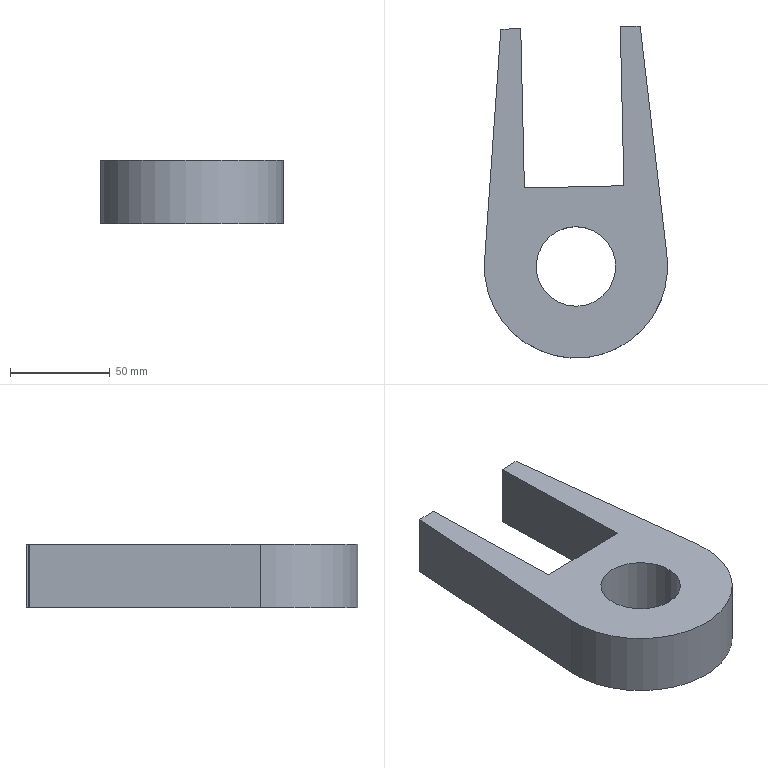Component | NX | 11 | 1 solid | 11 faces | box 92 x 166.77 x 32 mm | volume 249939 mm3 | plane 9 | cylinder 2 | commonest cylinder face diameters 92 x1 40 x1
STEP:
#1=CARTESIAN_POINT('',(0.,0.,0.));
#2=DIRECTION('',(0.,0.,1.));
#3=DIRECTION('',(1.,0.,0.));
#4=AXIS2_PLACEMENT_3D('',#1,#2,#3);
#5=CARTESIAN_POINT('',(-323.626,-1050.37,184.288));
#6=VERTEX_POINT('',#5);
#7=CARTESIAN_POINT('',(-313.628,-1050.142,184.288));
#8=VERTEX_POINT('',#7);
#9=CARTESIAN_POINT('',(-323.626,-1050.37,184.288));
#10=DIRECTION('',(0.9997,0.02285,0.));
#11=VECTOR('',#10,1.);
#12=LINE('',#9,#11);
#13=CARTESIAN_POINT('',(-323.626,-1050.37,152.288));
#14=DIRECTION('',(0.02285,-0.9997,0.));
#15=DIRECTION('',(-0.9997,-0.02285,0.));
#16=AXIS2_PLACEMENT_3D('',#13,#14,#15);
#17=PLANE('',#16);
#18=CARTESIAN_POINT('',(0.,-32.));
#19=DIRECTION('',(-1.,0.));
#20=VECTOR('',#19,1.);
#21=LINE('',#18,#20);
#22=(GEOMETRIC_REPRESENTATION_CONTEXT(2)PARAMETRIC_REPRESENTATION_CONTEXT()REPRESENTATION_CONTEXT('',''));
#23=DEFINITIONAL_REPRESENTATION('',(#21),#22);
#24=PCURVE('',#17,#23);
#25=CARTESIAN_POINT('',(-345.877,-1170.91,184.288));
#26=DIRECTION('',(0.,0.,-1.));
#27=DIRECTION('',(0.9997,0.02285,0.));
#28=AXIS2_PLACEMENT_3D('',#25,#26,#27);
#29=PLANE('',#28);
#30=CARTESIAN_POINT('',(25.,-120.));
#31=DIRECTION('',(1.,0.));
#32=VECTOR('',#31,1.);
#33=LINE('',#30,#32);
#34=(GEOMETRIC_REPRESENTATION_CONTEXT(2)PARAMETRIC_REPRESENTATION_CONTEXT()REPRESENTATION_CONTEXT('',''));
#35=DEFINITIONAL_REPRESENTATION('',(#33),#34);
#36=PCURVE('',#29,#35);
#37=SURFACE_CURVE('',#12,(#24,#36),.PCURVE_S1.);
#38=EDGE_CURVE('',#6,#8,#37,.T.);
#39=ORIENTED_EDGE('',*,*,#38,.T.);
#40=CARTESIAN_POINT('',(-313.628,-1050.142,152.288));
#41=VERTEX_POINT('',#40);
#42=CARTESIAN_POINT('',(-313.628,-1050.142,152.288));
#43=DIRECTION('',(0.,0.,1.));
#44=VECTOR('',#43,1.);
#45=LINE('',#42,#44);
#46=CARTESIAN_POINT('',(-10.,0.));
#47=DIRECTION('',(0.,-1.));
#48=VECTOR('',#47,1.);
#49=LINE('',#46,#48);
#50=(GEOMETRIC_REPRESENTATION_CONTEXT(2)PARAMETRIC_REPRESENTATION_CONTEXT()REPRESENTATION_CONTEXT('',''));
#51=DEFINITIONAL_REPRESENTATION('',(#49),#50);
#52=PCURVE('',#17,#51);
#53=CARTESIAN_POINT('',(-313.628,-1050.142,152.288));
#54=DIRECTION('',(-0.9933,-0.1157,0.));
#55=DIRECTION('',(-0.1157,0.9933,0.));
#56=AXIS2_PLACEMENT_3D('',#53,#54,#55);
#57=PLANE('',#56);
#58=CARTESIAN_POINT('',(0.,0.));
#59=DIRECTION('',(0.,-1.));
#60=VECTOR('',#59,1.);
#61=LINE('',#58,#60);
#62=(GEOMETRIC_REPRESENTATION_CONTEXT(2)PARAMETRIC_REPRESENTATION_CONTEXT()REPRESENTATION_CONTEXT('',''));
#63=DEFINITIONAL_REPRESENTATION('',(#61),#62);
#64=PCURVE('',#57,#63);
#65=SURFACE_CURVE('',#45,(#52,#64),.PCURVE_S1.);
#66=EDGE_CURVE('',#41,#8,#65,.T.);
#67=ORIENTED_EDGE('',*,*,#66,.F.);
#68=CARTESIAN_POINT('',(-323.626,-1050.37,152.288));
#69=VERTEX_POINT('',#68);
#70=CARTESIAN_POINT('',(-323.626,-1050.37,152.288));
#71=DIRECTION('',(0.9997,0.02285,0.));
#72=VECTOR('',#71,1.);
#73=LINE('',#70,#72);
#74=CARTESIAN_POINT('',(0.,0.));
#75=DIRECTION('',(-1.,0.));
#76=VECTOR('',#75,1.);
#77=LINE('',#74,#76);
#78=(GEOMETRIC_REPRESENTATION_CONTEXT(2)PARAMETRIC_REPRESENTATION_CONTEXT()REPRESENTATION_CONTEXT('',''));
#79=DEFINITIONAL_REPRESENTATION('',(#77),#78);
#80=PCURVE('',#17,#79);
#81=CARTESIAN_POINT('',(-345.877,-1170.91,152.288));
#82=DIRECTION('',(0.,0.,-1.));
#83=DIRECTION('',(0.9997,0.02285,0.));
#84=AXIS2_PLACEMENT_3D('',#81,#82,#83);
#85=PLANE('',#84);
#86=CARTESIAN_POINT('',(25.,-120.));
#87=DIRECTION('',(1.,0.));
#88=VECTOR('',#87,1.);
#89=LINE('',#86,#88);
#90=(GEOMETRIC_REPRESENTATION_CONTEXT(2)PARAMETRIC_REPRESENTATION_CONTEXT()REPRESENTATION_CONTEXT('',''));
#91=DEFINITIONAL_REPRESENTATION('',(#89),#90);
#92=PCURVE('',#85,#91);
#93=SURFACE_CURVE('',#73,(#80,#92),.PCURVE_S1.);
#94=EDGE_CURVE('',#69,#41,#93,.T.);
#95=ORIENTED_EDGE('',*,*,#94,.F.);
#96=CARTESIAN_POINT('',(-323.626,-1050.37,152.288));
#97=DIRECTION('',(0.,0.,1.));
#98=VECTOR('',#97,1.);
#99=LINE('',#96,#98);
#100=CARTESIAN_POINT('',(0.,0.));
#101=DIRECTION('',(0.,-1.));
#102=VECTOR('',#101,1.);
#103=LINE('',#100,#102);
#104=(GEOMETRIC_REPRESENTATION_CONTEXT(2)PARAMETRIC_REPRESENTATION_CONTEXT()REPRESENTATION_CONTEXT('',''));
#105=DEFINITIONAL_REPRESENTATION('',(#103),#104);
#106=PCURVE('',#17,#105);
#107=CARTESIAN_POINT('',(-321.797,-1130.349,152.288));
#108=DIRECTION('',(0.9997,0.02285,0.));
#109=DIRECTION('',(0.,0.,1.));
#110=AXIS2_PLACEMENT_3D('',#107,#108,#109);
#111=PLANE('',#110);
#112=CARTESIAN_POINT('',(0.,-80.));
#113=DIRECTION('',(1.,0.));
#114=VECTOR('',#113,1.);
#115=LINE('',#112,#114);
#116=(GEOMETRIC_REPRESENTATION_CONTEXT(2)PARAMETRIC_REPRESENTATION_CONTEXT()REPRESENTATION_CONTEXT('',''));
#117=DEFINITIONAL_REPRESENTATION('',(#115),#116);
#118=PCURVE('',#111,#117);
#119=SURFACE_CURVE('',#99,(#106,#118),.PCURVE_S1.);
#120=EDGE_CURVE('',#69,#6,#119,.T.);
#121=ORIENTED_EDGE('',*,*,#120,.T.);
#122=EDGE_LOOP('',(#39,#67,#95,#121));
#123=FACE_BOUND('',#122,.T.);
#124=ADVANCED_FACE('',(#123),#17,.F.);
#125=CARTESIAN_POINT('',(-300.185,-1165.59,184.288));
#126=VERTEX_POINT('',#125);
#127=CARTESIAN_POINT('',(-313.628,-1050.142,184.288));
#128=DIRECTION('',(0.1157,-0.9933,0.));
#129=VECTOR('',#128,1.);
#130=LINE('',#127,#129);
#131=CARTESIAN_POINT('',(0.,-32.));
#132=DIRECTION('',(-1.,0.));
#133=VECTOR('',#132,1.);
#134=LINE('',#131,#133);
#135=(GEOMETRIC_REPRESENTATION_CONTEXT(2)PARAMETRIC_REPRESENTATION_CONTEXT()REPRESENTATION_CONTEXT('',''));
#136=DEFINITIONAL_REPRESENTATION('',(#134),#135);
#137=PCURVE('',#57,#136);
#138=CARTESIAN_POINT('',(35.,-120.));
#139=DIRECTION('',(0.09293,0.9957));
#140=VECTOR('',#139,1.);
#141=LINE('',#138,#140);
#142=(GEOMETRIC_REPRESENTATION_CONTEXT(2)PARAMETRIC_REPRESENTATION_CONTEXT()REPRESENTATION_CONTEXT('',''));
#143=DEFINITIONAL_REPRESENTATION('',(#141),#142);
#144=PCURVE('',#29,#143);
#145=SURFACE_CURVE('',#130,(#137,#144),.PCURVE_S1.);
#146=EDGE_CURVE('',#8,#126,#145,.T.);
#147=ORIENTED_EDGE('',*,*,#146,.T.);
#148=CARTESIAN_POINT('',(-300.185,-1165.59,152.288));
#149=VERTEX_POINT('',#148);
#150=CARTESIAN_POINT('',(-300.185,-1165.59,152.288));
#151=DIRECTION('',(0.,0.,1.));
#152=VECTOR('',#151,1.);
#153=LINE('',#150,#152);
#154=CARTESIAN_POINT('',(-116.228,0.));
#155=DIRECTION('',(0.,-1.));
#156=VECTOR('',#155,1.);
#157=LINE('',#154,#156);
#158=(GEOMETRIC_REPRESENTATION_CONTEXT(2)PARAMETRIC_REPRESENTATION_CONTEXT()REPRESENTATION_CONTEXT('',''));
#159=DEFINITIONAL_REPRESENTATION('',(#157),#158);
#160=PCURVE('',#57,#159);
#161=CARTESIAN_POINT('',(-345.877,-1170.91,152.288));
#162=DIRECTION('',(0.,0.,1.));
#163=DIRECTION('',(-0.9997,-0.02285,0.));
#164=AXIS2_PLACEMENT_3D('',#161,#162,#163);
#165=CYLINDRICAL_SURFACE('',#164,46.);
#166=CARTESIAN_POINT('',(3.235,0.));
#167=DIRECTION('',(0.,1.));
#168=VECTOR('',#167,1.);
#169=LINE('',#166,#168);
#170=(GEOMETRIC_REPRESENTATION_CONTEXT(2)PARAMETRIC_REPRESENTATION_CONTEXT()REPRESENTATION_CONTEXT('',''));
#171=DEFINITIONAL_REPRESENTATION('',(#169),#170);
#172=PCURVE('',#165,#171);
#173=SURFACE_CURVE('',#153,(#160,#172),.PCURVE_S1.);
#174=EDGE_CURVE('',#149,#126,#173,.T.);
#175=ORIENTED_EDGE('',*,*,#174,.F.);
#176=CARTESIAN_POINT('',(-313.628,-1050.142,152.288));
#177=DIRECTION('',(0.1157,-0.9933,0.));
#178=VECTOR('',#177,1.);
#179=LINE('',#176,#178);
#180=CARTESIAN_POINT('',(0.,0.));
#181=DIRECTION('',(-1.,0.));
#182=VECTOR('',#181,1.);
#183=LINE('',#180,#182);
#184=(GEOMETRIC_REPRESENTATION_CONTEXT(2)PARAMETRIC_REPRESENTATION_CONTEXT()REPRESENTATION_CONTEXT('',''));
#185=DEFINITIONAL_REPRESENTATION('',(#183),#184);
#186=PCURVE('',#57,#185);
#187=CARTESIAN_POINT('',(35.,-120.));
#188=DIRECTION('',(0.09293,0.9957));
#189=VECTOR('',#188,1.);
#190=LINE('',#187,#189);
#191=(GEOMETRIC_REPRESENTATION_CONTEXT(2)PARAMETRIC_REPRESENTATION_CONTEXT()REPRESENTATION_CONTEXT('',''));
#192=DEFINITIONAL_REPRESENTATION('',(#190),#191);
#193=PCURVE('',#85,#192);
#194=SURFACE_CURVE('',#179,(#186,#193),.PCURVE_S1.);
#195=EDGE_CURVE('',#41,#149,#194,.T.);
#196=ORIENTED_EDGE('',*,*,#195,.F.);
#197=ORIENTED_EDGE('',*,*,#66,.T.);
#198=EDGE_LOOP('',(#147,#175,#196,#197));
#199=FACE_BOUND('',#198,.T.);
#200=ADVANCED_FACE('',(#199),#57,.F.);
#201=CARTESIAN_POINT('',(-391.763,-1167.683,184.288));
#202=VERTEX_POINT('',#201);
#203=CARTESIAN_POINT('',(-345.877,-1170.91,184.288));
#204=DIRECTION('',(0.,0.,-1.));
#205=DIRECTION('',(0.02285,-0.9997,0.));
#206=AXIS2_PLACEMENT_3D('',#203,#204,#205);
#207=CIRCLE('',#206,46.);
#208=CARTESIAN_POINT('',(7.854,32.));
#209=DIRECTION('',(-1.,0.));
#210=VECTOR('',#209,1.);
#211=LINE('',#208,#210);
#212=(GEOMETRIC_REPRESENTATION_CONTEXT(2)PARAMETRIC_REPRESENTATION_CONTEXT()REPRESENTATION_CONTEXT('',''));
#213=DEFINITIONAL_REPRESENTATION('',(#211),#212);
#214=PCURVE('',#165,#213);
#215=CARTESIAN_POINT('',(0.,0.));
#216=DIRECTION('',(-0.,1.));
#217=AXIS2_PLACEMENT_2D('',#215,#216);
#218=CIRCLE('',#217,46.);
#219=(GEOMETRIC_REPRESENTATION_CONTEXT(2)PARAMETRIC_REPRESENTATION_CONTEXT()REPRESENTATION_CONTEXT('',''));
#220=DEFINITIONAL_REPRESENTATION('',(#218),#219);
#221=PCURVE('',#29,#220);
#222=SURFACE_CURVE('',#207,(#214,#221),.PCURVE_S1.);
#223=EDGE_CURVE('',#126,#202,#222,.T.);
#224=ORIENTED_EDGE('',*,*,#223,.T.);
#225=CARTESIAN_POINT('',(-391.763,-1167.683,152.288));
#226=VERTEX_POINT('',#225);
#227=CARTESIAN_POINT('',(-391.763,-1167.683,152.288));
#228=DIRECTION('',(0.,0.,1.));
#229=VECTOR('',#228,1.);
#230=LINE('',#227,#229);
#231=CARTESIAN_POINT('',(-0.09306,0.));
#232=DIRECTION('',(0.,1.));
#233=VECTOR('',#232,1.);
#234=LINE('',#231,#233);
#235=(GEOMETRIC_REPRESENTATION_CONTEXT(2)PARAMETRIC_REPRESENTATION_CONTEXT()REPRESENTATION_CONTEXT('',''));
#236=DEFINITIONAL_REPRESENTATION('',(#234),#235);
#237=PCURVE('',#165,#236);
#238=CARTESIAN_POINT('',(-391.763,-1167.683,152.288));
#239=DIRECTION('',(0.9975,-0.07015,0.));
#240=DIRECTION('',(-0.07015,-0.9975,0.));
#241=AXIS2_PLACEMENT_3D('',#238,#239,#240);
#242=PLANE('',#241);
#243=CARTESIAN_POINT('',(0.,0.));
#244=DIRECTION('',(0.,-1.));
#245=VECTOR('',#244,1.);
#246=LINE('',#243,#245);
#247=(GEOMETRIC_REPRESENTATION_CONTEXT(2)PARAMETRIC_REPRESENTATION_CONTEXT()REPRESENTATION_CONTEXT('',''));
#248=DEFINITIONAL_REPRESENTATION('',(#246),#247);
#249=PCURVE('',#242,#248);
#250=SURFACE_CURVE('',#230,(#237,#249),.PCURVE_S1.);
#251=EDGE_CURVE('',#226,#202,#250,.T.);
#252=ORIENTED_EDGE('',*,*,#251,.F.);
#253=CARTESIAN_POINT('',(-345.877,-1170.91,152.288));
#254=DIRECTION('',(0.,0.,-1.));
#255=DIRECTION('',(0.02285,-0.9997,0.));
#256=AXIS2_PLACEMENT_3D('',#253,#254,#255);
#257=CIRCLE('',#256,46.);
#258=CARTESIAN_POINT('',(7.854,0.));
#259=DIRECTION('',(-1.,0.));
#260=VECTOR('',#259,1.);
#261=LINE('',#258,#260);
#262=(GEOMETRIC_REPRESENTATION_CONTEXT(2)PARAMETRIC_REPRESENTATION_CONTEXT()REPRESENTATION_CONTEXT('',''));
#263=DEFINITIONAL_REPRESENTATION('',(#261),#262);
#264=PCURVE('',#165,#263);
#265=CARTESIAN_POINT('',(0.,0.));
#266=DIRECTION('',(-0.,1.));
#267=AXIS2_PLACEMENT_2D('',#265,#266);
#268=CIRCLE('',#267,46.);
#269=(GEOMETRIC_REPRESENTATION_CONTEXT(2)PARAMETRIC_REPRESENTATION_CONTEXT()REPRESENTATION_CONTEXT('',''));
#270=DEFINITIONAL_REPRESENTATION('',(#268),#269);
#271=PCURVE('',#85,#270);
#272=SURFACE_CURVE('',#257,(#264,#271),.PCURVE_S1.);
#273=EDGE_CURVE('',#149,#226,#272,.T.);
#274=ORIENTED_EDGE('',*,*,#273,.F.);
#275=ORIENTED_EDGE('',*,*,#174,.T.);
#276=EDGE_LOOP('',(#224,#252,#274,#275));
#277=FACE_BOUND('',#276,.T.);
#278=ADVANCED_FACE('',(#277),#165,.T.);
#279=CARTESIAN_POINT('',(-383.61,-1051.742,184.288));
#280=VERTEX_POINT('',#279);
#281=CARTESIAN_POINT('',(-391.763,-1167.683,184.288));
#282=DIRECTION('',(0.07015,0.9975,0.));
#283=VECTOR('',#282,1.);
#284=LINE('',#281,#283);
#285=CARTESIAN_POINT('',(0.,-32.));
#286=DIRECTION('',(-1.,0.));
#287=VECTOR('',#286,1.);
#288=LINE('',#285,#287);
#289=(GEOMETRIC_REPRESENTATION_CONTEXT(2)PARAMETRIC_REPRESENTATION_CONTEXT()REPRESENTATION_CONTEXT('',''));
#290=DEFINITIONAL_REPRESENTATION('',(#288),#289);
#291=PCURVE('',#242,#290);
#292=CARTESIAN_POINT('',(-45.801,-4.275));
#293=DIRECTION('',(0.09293,-0.9957));
#294=VECTOR('',#293,1.);
#295=LINE('',#292,#294);
#296=(GEOMETRIC_REPRESENTATION_CONTEXT(2)PARAMETRIC_REPRESENTATION_CONTEXT()REPRESENTATION_CONTEXT('',''));
#297=DEFINITIONAL_REPRESENTATION('',(#295),#296);
#298=PCURVE('',#29,#297);
#299=SURFACE_CURVE('',#284,(#291,#298),.PCURVE_S1.);
#300=EDGE_CURVE('',#202,#280,#299,.T.);
#301=ORIENTED_EDGE('',*,*,#300,.T.);
#302=CARTESIAN_POINT('',(-383.61,-1051.742,152.288));
#303=VERTEX_POINT('',#302);
#304=CARTESIAN_POINT('',(-383.61,-1051.742,152.288));
#305=DIRECTION('',(0.,0.,1.));
#306=VECTOR('',#305,1.);
#307=LINE('',#304,#306);
#308=CARTESIAN_POINT('',(-116.228,0.));
#309=DIRECTION('',(0.,-1.));
#310=VECTOR('',#309,1.);
#311=LINE('',#308,#310);
#312=(GEOMETRIC_REPRESENTATION_CONTEXT(2)PARAMETRIC_REPRESENTATION_CONTEXT()REPRESENTATION_CONTEXT('',''));
#313=DEFINITIONAL_REPRESENTATION('',(#311),#312);
#314=PCURVE('',#242,#313);
#315=CARTESIAN_POINT('',(-383.61,-1051.742,152.288));
#316=DIRECTION('',(0.02285,-0.9997,0.));
#317=DIRECTION('',(-0.9997,-0.02285,0.));
#318=AXIS2_PLACEMENT_3D('',#315,#316,#317);
#319=PLANE('',#318);
#320=CARTESIAN_POINT('',(0.,0.));
#321=DIRECTION('',(0.,-1.));
#322=VECTOR('',#321,1.);
#323=LINE('',#320,#322);
#324=(GEOMETRIC_REPRESENTATION_CONTEXT(2)PARAMETRIC_REPRESENTATION_CONTEXT()REPRESENTATION_CONTEXT('',''));
#325=DEFINITIONAL_REPRESENTATION('',(#323),#324);
#326=PCURVE('',#319,#325);
#327=SURFACE_CURVE('',#307,(#314,#326),.PCURVE_S1.);
#328=EDGE_CURVE('',#303,#280,#327,.T.);
#329=ORIENTED_EDGE('',*,*,#328,.F.);
#330=CARTESIAN_POINT('',(-391.763,-1167.683,152.288));
#331=DIRECTION('',(0.07015,0.9975,0.));
#332=VECTOR('',#331,1.);
#333=LINE('',#330,#332);
#334=CARTESIAN_POINT('',(0.,0.));
#335=DIRECTION('',(-1.,0.));
#336=VECTOR('',#335,1.);
#337=LINE('',#334,#336);
#338=(GEOMETRIC_REPRESENTATION_CONTEXT(2)PARAMETRIC_REPRESENTATION_CONTEXT()REPRESENTATION_CONTEXT('',''));
#339=DEFINITIONAL_REPRESENTATION('',(#337),#338);
#340=PCURVE('',#242,#339);
#341=CARTESIAN_POINT('',(-45.801,-4.275));
#342=DIRECTION('',(0.09293,-0.9957));
#343=VECTOR('',#342,1.);
#344=LINE('',#341,#343);
#345=(GEOMETRIC_REPRESENTATION_CONTEXT(2)PARAMETRIC_REPRESENTATION_CONTEXT()REPRESENTATION_CONTEXT('',''));
#346=DEFINITIONAL_REPRESENTATION('',(#344),#345);
#347=PCURVE('',#85,#346);
#348=SURFACE_CURVE('',#333,(#340,#347),.PCURVE_S1.);
#349=EDGE_CURVE('',#226,#303,#348,.T.);
#350=ORIENTED_EDGE('',*,*,#349,.F.);
#351=ORIENTED_EDGE('',*,*,#251,.T.);
#352=EDGE_LOOP('',(#301,#329,#350,#351));
#353=FACE_BOUND('',#352,.T.);
#354=ADVANCED_FACE('',(#353),#242,.F.);
#355=CARTESIAN_POINT('',(-373.613,-1051.513,184.288));
#356=VERTEX_POINT('',#355);
#357=CARTESIAN_POINT('',(-383.61,-1051.742,184.288));
#358=DIRECTION('',(0.9997,0.02285,0.));
#359=VECTOR('',#358,1.);
#360=LINE('',#357,#359);
#361=CARTESIAN_POINT('',(0.,-32.));
#362=DIRECTION('',(-1.,0.));
#363=VECTOR('',#362,1.);
#364=LINE('',#361,#363);
#365=(GEOMETRIC_REPRESENTATION_CONTEXT(2)PARAMETRIC_REPRESENTATION_CONTEXT()REPRESENTATION_CONTEXT('',''));
#366=DEFINITIONAL_REPRESENTATION('',(#364),#365);
#367=PCURVE('',#319,#366);
#368=CARTESIAN_POINT('',(-35.,-120.));
#369=DIRECTION('',(1.,0.));
#370=VECTOR('',#369,1.);
#371=LINE('',#368,#370);
#372=(GEOMETRIC_REPRESENTATION_CONTEXT(2)PARAMETRIC_REPRESENTATION_CONTEXT()REPRESENTATION_CONTEXT('',''));
#373=DEFINITIONAL_REPRESENTATION('',(#371),#372);
#374=PCURVE('',#29,#373);
#375=SURFACE_CURVE('',#360,(#367,#374),.PCURVE_S1.);
#376=EDGE_CURVE('',#280,#356,#375,.T.);
#377=ORIENTED_EDGE('',*,*,#376,.T.);
#378=CARTESIAN_POINT('',(-373.613,-1051.513,152.288));
#379=VERTEX_POINT('',#378);
#380=CARTESIAN_POINT('',(-373.613,-1051.513,152.288));
#381=DIRECTION('',(0.,0.,1.));
#382=VECTOR('',#381,1.);
#383=LINE('',#380,#382);
#384=CARTESIAN_POINT('',(-10.,0.));
#385=DIRECTION('',(0.,-1.));
#386=VECTOR('',#385,1.);
#387=LINE('',#384,#386);
#388=(GEOMETRIC_REPRESENTATION_CONTEXT(2)PARAMETRIC_REPRESENTATION_CONTEXT()REPRESENTATION_CONTEXT('',''));
#389=DEFINITIONAL_REPRESENTATION('',(#387),#388);
#390=PCURVE('',#319,#389);
#391=CARTESIAN_POINT('',(-373.613,-1051.513,152.288));
#392=DIRECTION('',(-0.9997,-0.02285,0.));
#393=DIRECTION('',(0.,0.,-1.));
#394=AXIS2_PLACEMENT_3D('',#391,#392,#393);
#395=PLANE('',#394);
#396=CARTESIAN_POINT('',(0.,0.));
#397=DIRECTION('',(-1.,0.));
#398=VECTOR('',#397,1.);
#399=LINE('',#396,#398);
#400=(GEOMETRIC_REPRESENTATION_CONTEXT(2)PARAMETRIC_REPRESENTATION_CONTEXT()REPRESENTATION_CONTEXT('',''));
#401=DEFINITIONAL_REPRESENTATION('',(#399),#400);
#402=PCURVE('',#395,#401);
#403=SURFACE_CURVE('',#383,(#390,#402),.PCURVE_S1.);
#404=EDGE_CURVE('',#379,#356,#403,.T.);
#405=ORIENTED_EDGE('',*,*,#404,.F.);
#406=CARTESIAN_POINT('',(-383.61,-1051.742,152.288));
#407=DIRECTION('',(0.9997,0.02285,0.));
#408=VECTOR('',#407,1.);
#409=LINE('',#406,#408);
#410=CARTESIAN_POINT('',(0.,0.));
#411=DIRECTION('',(-1.,0.));
#412=VECTOR('',#411,1.);
#413=LINE('',#410,#412);
#414=(GEOMETRIC_REPRESENTATION_CONTEXT(2)PARAMETRIC_REPRESENTATION_CONTEXT()REPRESENTATION_CONTEXT('',''));
#415=DEFINITIONAL_REPRESENTATION('',(#413),#414);
#416=PCURVE('',#319,#415);
#417=CARTESIAN_POINT('',(-35.,-120.));
#418=DIRECTION('',(1.,0.));
#419=VECTOR('',#418,1.);
#420=LINE('',#417,#419);
#421=(GEOMETRIC_REPRESENTATION_CONTEXT(2)PARAMETRIC_REPRESENTATION_CONTEXT()REPRESENTATION_CONTEXT('',''));
#422=DEFINITIONAL_REPRESENTATION('',(#420),#421);
#423=PCURVE('',#85,#422);
#424=SURFACE_CURVE('',#409,(#416,#423),.PCURVE_S1.);
#425=EDGE_CURVE('',#303,#379,#424,.T.);
#426=ORIENTED_EDGE('',*,*,#425,.F.);
#427=ORIENTED_EDGE('',*,*,#328,.T.);
#428=EDGE_LOOP('',(#377,#405,#426,#427));
#429=FACE_BOUND('',#428,.T.);
#430=ADVANCED_FACE('',(#429),#319,.F.);
#431=CARTESIAN_POINT('',(-371.784,-1131.492,184.288));
#432=VERTEX_POINT('',#431);
#433=CARTESIAN_POINT('',(-373.613,-1051.513,184.288));
#434=DIRECTION('',(0.02285,-0.9997,0.));
#435=VECTOR('',#434,1.);
#436=LINE('',#433,#435);
#437=CARTESIAN_POINT('',(-32.,0.));
#438=DIRECTION('',(0.,1.));
#439=VECTOR('',#438,1.);
#440=LINE('',#437,#439);
#441=(GEOMETRIC_REPRESENTATION_CONTEXT(2)PARAMETRIC_REPRESENTATION_CONTEXT()REPRESENTATION_CONTEXT('',''));
#442=DEFINITIONAL_REPRESENTATION('',(#440),#441);
#443=PCURVE('',#395,#442);
#444=CARTESIAN_POINT('',(-25.,-120.));
#445=DIRECTION('',(0.,1.));
#446=VECTOR('',#445,1.);
#447=LINE('',#444,#446);
#448=(GEOMETRIC_REPRESENTATION_CONTEXT(2)PARAMETRIC_REPRESENTATION_CONTEXT()REPRESENTATION_CONTEXT('',''));
#449=DEFINITIONAL_REPRESENTATION('',(#447),#448);
#450=PCURVE('',#29,#449);
#451=SURFACE_CURVE('',#436,(#443,#450),.PCURVE_S1.);
#452=EDGE_CURVE('',#356,#432,#451,.T.);
#453=ORIENTED_EDGE('',*,*,#452,.T.);
#454=CARTESIAN_POINT('',(-371.784,-1131.492,152.288));
#455=VERTEX_POINT('',#454);
#456=CARTESIAN_POINT('',(-371.784,-1131.492,152.288));
#457=DIRECTION('',(0.,0.,1.));
#458=VECTOR('',#457,1.);
#459=LINE('',#456,#458);
#460=CARTESIAN_POINT('',(0.,80.));
#461=DIRECTION('',(-1.,0.));
#462=VECTOR('',#461,1.);
#463=LINE('',#460,#462);
#464=(GEOMETRIC_REPRESENTATION_CONTEXT(2)PARAMETRIC_REPRESENTATION_CONTEXT()REPRESENTATION_CONTEXT('',''));
#465=DEFINITIONAL_REPRESENTATION('',(#463),#464);
#466=PCURVE('',#395,#465);
#467=CARTESIAN_POINT('',(-371.784,-1131.492,152.288));
#468=DIRECTION('',(0.02285,-0.9997,0.));
#469=DIRECTION('',(-0.9997,-0.02285,0.));
#470=AXIS2_PLACEMENT_3D('',#467,#468,#469);
#471=PLANE('',#470);
#472=CARTESIAN_POINT('',(0.,0.));
#473=DIRECTION('',(0.,-1.));
#474=VECTOR('',#473,1.);
#475=LINE('',#472,#474);
#476=(GEOMETRIC_REPRESENTATION_CONTEXT(2)PARAMETRIC_REPRESENTATION_CONTEXT()REPRESENTATION_CONTEXT('',''));
#477=DEFINITIONAL_REPRESENTATION('',(#475),#476);
#478=PCURVE('',#471,#477);
#479=SURFACE_CURVE('',#459,(#466,#478),.PCURVE_S1.);
#480=EDGE_CURVE('',#455,#432,#479,.T.);
#481=ORIENTED_EDGE('',*,*,#480,.F.);
#482=CARTESIAN_POINT('',(-373.613,-1051.513,152.288));
#483=DIRECTION('',(0.02285,-0.9997,0.));
#484=VECTOR('',#483,1.);
#485=LINE('',#482,#484);
#486=CARTESIAN_POINT('',(0.,0.));
#487=DIRECTION('',(0.,1.));
#488=VECTOR('',#487,1.);
#489=LINE('',#486,#488);
#490=(GEOMETRIC_REPRESENTATION_CONTEXT(2)PARAMETRIC_REPRESENTATION_CONTEXT()REPRESENTATION_CONTEXT('',''));
#491=DEFINITIONAL_REPRESENTATION('',(#489),#490);
#492=PCURVE('',#395,#491);
#493=CARTESIAN_POINT('',(-25.,-120.));
#494=DIRECTION('',(0.,1.));
#495=VECTOR('',#494,1.);
#496=LINE('',#493,#495);
#497=(GEOMETRIC_REPRESENTATION_CONTEXT(2)PARAMETRIC_REPRESENTATION_CONTEXT()REPRESENTATION_CONTEXT('',''));
#498=DEFINITIONAL_REPRESENTATION('',(#496),#497);
#499=PCURVE('',#85,#498);
#500=SURFACE_CURVE('',#485,(#492,#499),.PCURVE_S1.);
#501=EDGE_CURVE('',#379,#455,#500,.T.);
#502=ORIENTED_EDGE('',*,*,#501,.F.);
#503=ORIENTED_EDGE('',*,*,#404,.T.);
#504=EDGE_LOOP('',(#453,#481,#502,#503));
#505=FACE_BOUND('',#504,.T.);
#506=ADVANCED_FACE('',(#505),#395,.F.);
#507=CARTESIAN_POINT('',(-321.797,-1130.349,184.288));
#508=VERTEX_POINT('',#507);
#509=CARTESIAN_POINT('',(-371.784,-1131.492,184.288));
#510=DIRECTION('',(0.9997,0.02285,0.));
#511=VECTOR('',#510,1.);
#512=LINE('',#509,#511);
#513=CARTESIAN_POINT('',(0.,-32.));
#514=DIRECTION('',(-1.,0.));
#515=VECTOR('',#514,1.);
#516=LINE('',#513,#515);
#517=(GEOMETRIC_REPRESENTATION_CONTEXT(2)PARAMETRIC_REPRESENTATION_CONTEXT()REPRESENTATION_CONTEXT('',''));
#518=DEFINITIONAL_REPRESENTATION('',(#516),#517);
#519=PCURVE('',#471,#518);
#520=CARTESIAN_POINT('',(-25.,-40.));
#521=DIRECTION('',(1.,0.));
#522=VECTOR('',#521,1.);
#523=LINE('',#520,#522);
#524=(GEOMETRIC_REPRESENTATION_CONTEXT(2)PARAMETRIC_REPRESENTATION_CONTEXT()REPRESENTATION_CONTEXT('',''));
#525=DEFINITIONAL_REPRESENTATION('',(#523),#524);
#526=PCURVE('',#29,#525);
#527=SURFACE_CURVE('',#512,(#519,#526),.PCURVE_S1.);
#528=EDGE_CURVE('',#432,#508,#527,.T.);
#529=ORIENTED_EDGE('',*,*,#528,.T.);
#530=CARTESIAN_POINT('',(-321.797,-1130.349,152.288));
#531=VERTEX_POINT('',#530);
#532=CARTESIAN_POINT('',(-321.797,-1130.349,152.288));
#533=DIRECTION('',(0.,0.,1.));
#534=VECTOR('',#533,1.);
#535=LINE('',#532,#534);
#536=CARTESIAN_POINT('',(-50.,0.));
#537=DIRECTION('',(0.,-1.));
#538=VECTOR('',#537,1.);
#539=LINE('',#536,#538);
#540=(GEOMETRIC_REPRESENTATION_CONTEXT(2)PARAMETRIC_REPRESENTATION_CONTEXT()REPRESENTATION_CONTEXT('',''));
#541=DEFINITIONAL_REPRESENTATION('',(#539),#540);
#542=PCURVE('',#471,#541);
#543=CARTESIAN_POINT('',(0.,0.));
#544=DIRECTION('',(1.,0.));
#545=VECTOR('',#544,1.);
#546=LINE('',#543,#545);
#547=(GEOMETRIC_REPRESENTATION_CONTEXT(2)PARAMETRIC_REPRESENTATION_CONTEXT()REPRESENTATION_CONTEXT('',''));
#548=DEFINITIONAL_REPRESENTATION('',(#546),#547);
#549=PCURVE('',#111,#548);
#550=SURFACE_CURVE('',#535,(#542,#549),.PCURVE_S1.);
#551=EDGE_CURVE('',#531,#508,#550,.T.);
#552=ORIENTED_EDGE('',*,*,#551,.F.);
#553=CARTESIAN_POINT('',(-371.784,-1131.492,152.288));
#554=DIRECTION('',(0.9997,0.02285,0.));
#555=VECTOR('',#554,1.);
#556=LINE('',#553,#555);
#557=CARTESIAN_POINT('',(0.,0.));
#558=DIRECTION('',(-1.,0.));
#559=VECTOR('',#558,1.);
#560=LINE('',#557,#559);
#561=(GEOMETRIC_REPRESENTATION_CONTEXT(2)PARAMETRIC_REPRESENTATION_CONTEXT()REPRESENTATION_CONTEXT('',''));
#562=DEFINITIONAL_REPRESENTATION('',(#560),#561);
#563=PCURVE('',#471,#562);
#564=CARTESIAN_POINT('',(-25.,-40.));
#565=DIRECTION('',(1.,0.));
#566=VECTOR('',#565,1.);
#567=LINE('',#564,#566);
#568=(GEOMETRIC_REPRESENTATION_CONTEXT(2)PARAMETRIC_REPRESENTATION_CONTEXT()REPRESENTATION_CONTEXT('',''));
#569=DEFINITIONAL_REPRESENTATION('',(#567),#568);
#570=PCURVE('',#85,#569);
#571=SURFACE_CURVE('',#556,(#563,#570),.PCURVE_S1.);
#572=EDGE_CURVE('',#455,#531,#571,.T.);
#573=ORIENTED_EDGE('',*,*,#572,.F.);
#574=ORIENTED_EDGE('',*,*,#480,.T.);
#575=EDGE_LOOP('',(#529,#552,#573,#574));
#576=FACE_BOUND('',#575,.T.);
#577=ADVANCED_FACE('',(#576),#471,.F.);
#578=CARTESIAN_POINT('',(-321.797,-1130.349,184.288));
#579=DIRECTION('',(-0.02285,0.9997,0.));
#580=VECTOR('',#579,1.);
#581=LINE('',#578,#580);
#582=CARTESIAN_POINT('',(32.,0.));
#583=DIRECTION('',(0.,-1.));
#584=VECTOR('',#583,1.);
#585=LINE('',#582,#584);
#586=(GEOMETRIC_REPRESENTATION_CONTEXT(2)PARAMETRIC_REPRESENTATION_CONTEXT()REPRESENTATION_CONTEXT('',''));
#587=DEFINITIONAL_REPRESENTATION('',(#585),#586);
#588=PCURVE('',#111,#587);
#589=CARTESIAN_POINT('',(25.,-40.));
#590=DIRECTION('',(0.,-1.));
#591=VECTOR('',#590,1.);
#592=LINE('',#589,#591);
#593=(GEOMETRIC_REPRESENTATION_CONTEXT(2)PARAMETRIC_REPRESENTATION_CONTEXT()REPRESENTATION_CONTEXT('',''));
#594=DEFINITIONAL_REPRESENTATION('',(#592),#593);
#595=PCURVE('',#29,#594);
#596=SURFACE_CURVE('',#581,(#588,#595),.PCURVE_S1.);
#597=EDGE_CURVE('',#508,#6,#596,.T.);
#598=ORIENTED_EDGE('',*,*,#597,.T.);
#599=ORIENTED_EDGE('',*,*,#120,.F.);
#600=CARTESIAN_POINT('',(-321.797,-1130.349,152.288));
#601=DIRECTION('',(-0.02285,0.9997,0.));
#602=VECTOR('',#601,1.);
#603=LINE('',#600,#602);
#604=CARTESIAN_POINT('',(0.,0.));
#605=DIRECTION('',(0.,-1.));
#606=VECTOR('',#605,1.);
#607=LINE('',#604,#606);
#608=(GEOMETRIC_REPRESENTATION_CONTEXT(2)PARAMETRIC_REPRESENTATION_CONTEXT()REPRESENTATION_CONTEXT('',''));
#609=DEFINITIONAL_REPRESENTATION('',(#607),#608);
#610=PCURVE('',#111,#609);
#611=CARTESIAN_POINT('',(25.,-40.));
#612=DIRECTION('',(0.,-1.));
#613=VECTOR('',#612,1.);
#614=LINE('',#611,#613);
#615=(GEOMETRIC_REPRESENTATION_CONTEXT(2)PARAMETRIC_REPRESENTATION_CONTEXT()REPRESENTATION_CONTEXT('',''));
#616=DEFINITIONAL_REPRESENTATION('',(#614),#615);
#617=PCURVE('',#85,#616);
#618=SURFACE_CURVE('',#603,(#610,#617),.PCURVE_S1.);
#619=EDGE_CURVE('',#531,#69,#618,.T.);
#620=ORIENTED_EDGE('',*,*,#619,.F.);
#621=ORIENTED_EDGE('',*,*,#551,.T.);
#622=EDGE_LOOP('',(#598,#599,#620,#621));
#623=FACE_BOUND('',#622,.T.);
#624=ADVANCED_FACE('',(#623),#111,.F.);
#625=CARTESIAN_POINT('',(-345.42,-1190.905,152.288));
#626=VERTEX_POINT('',#625);
#627=CARTESIAN_POINT('',(-345.877,-1170.91,152.288));
#628=DIRECTION('',(0.,0.,-1.));
#629=DIRECTION('',(0.02285,-0.9997,0.));
#630=AXIS2_PLACEMENT_3D('',#627,#628,#629);
#631=CIRCLE('',#630,20.);
#632=CARTESIAN_POINT('',(-345.877,-1170.91,152.288));
#633=DIRECTION('',(0.,0.,1.));
#634=DIRECTION('',(-0.9997,-0.02285,0.));
#635=AXIS2_PLACEMENT_3D('',#632,#633,#634);
#636=CYLINDRICAL_SURFACE('',#635,20.);
#637=CARTESIAN_POINT('',(7.854,0.));
#638=DIRECTION('',(-1.,0.));
#639=VECTOR('',#638,1.);
#640=LINE('',#637,#639);
#641=(GEOMETRIC_REPRESENTATION_CONTEXT(2)PARAMETRIC_REPRESENTATION_CONTEXT()REPRESENTATION_CONTEXT('',''));
#642=DEFINITIONAL_REPRESENTATION('',(#640),#641);
#643=PCURVE('',#636,#642);
#644=CARTESIAN_POINT('',(0.,0.));
#645=DIRECTION('',(-0.,1.));
#646=AXIS2_PLACEMENT_2D('',#644,#645);
#647=CIRCLE('',#646,20.);
#648=(GEOMETRIC_REPRESENTATION_CONTEXT(2)PARAMETRIC_REPRESENTATION_CONTEXT()REPRESENTATION_CONTEXT('',''));
#649=DEFINITIONAL_REPRESENTATION('',(#647),#648);
#650=PCURVE('',#85,#649);
#651=SURFACE_CURVE('',#631,(#643,#650),.PCURVE_S1.);
#652=EDGE_CURVE('',#626,#626,#651,.T.);
#653=ORIENTED_EDGE('',*,*,#652,.F.);
#654=CARTESIAN_POINT('',(-345.42,-1190.905,184.288));
#655=VERTEX_POINT('',#654);
#656=CARTESIAN_POINT('',(-345.42,-1190.905,152.288));
#657=CARTESIAN_POINT('',(-345.42,-1190.905,184.288));
#658=B_SPLINE_CURVE_WITH_KNOTS('',1,(#656,#657),.UNSPECIFIED.,.F.,.F.,(2,2),(0.,32.),.PIECEWISE_BEZIER_KNOTS.);
#659=CARTESIAN_POINT('',(7.854,0.));
#660=DIRECTION('',(0.,1.));
#661=VECTOR('',#660,1.);
#662=LINE('',#659,#661);
#663=(GEOMETRIC_REPRESENTATION_CONTEXT(2)PARAMETRIC_REPRESENTATION_CONTEXT()REPRESENTATION_CONTEXT('',''));
#664=DEFINITIONAL_REPRESENTATION('',(#662),#663);
#665=PCURVE('',#636,#664);
#666=CARTESIAN_POINT('',(1.571,0.));
#667=DIRECTION('',(0.,1.));
#668=VECTOR('',#667,1.);
#669=LINE('',#666,#668);
#670=(GEOMETRIC_REPRESENTATION_CONTEXT(2)PARAMETRIC_REPRESENTATION_CONTEXT()REPRESENTATION_CONTEXT('',''));
#671=DEFINITIONAL_REPRESENTATION('',(#669),#670);
#672=PCURVE('',#636,#671);
#673=SEAM_CURVE('',#658,(#665,#672),.PCURVE_S1.);
#674=EDGE_CURVE('',#626,#655,#673,.T.);
#675=ORIENTED_EDGE('',*,*,#674,.T.);
#676=CARTESIAN_POINT('',(-345.877,-1170.91,184.288));
#677=DIRECTION('',(0.,0.,-1.));
#678=DIRECTION('',(0.02285,-0.9997,0.));
#679=AXIS2_PLACEMENT_3D('',#676,#677,#678);
#680=CIRCLE('',#679,20.);
#681=CARTESIAN_POINT('',(7.854,32.));
#682=DIRECTION('',(-1.,0.));
#683=VECTOR('',#682,1.);
#684=LINE('',#681,#683);
#685=(GEOMETRIC_REPRESENTATION_CONTEXT(2)PARAMETRIC_REPRESENTATION_CONTEXT()REPRESENTATION_CONTEXT('',''));
#686=DEFINITIONAL_REPRESENTATION('',(#684),#685);
#687=PCURVE('',#636,#686);
#688=CARTESIAN_POINT('',(0.,0.));
#689=DIRECTION('',(-0.,1.));
#690=AXIS2_PLACEMENT_2D('',#688,#689);
#691=CIRCLE('',#690,20.);
#692=(GEOMETRIC_REPRESENTATION_CONTEXT(2)PARAMETRIC_REPRESENTATION_CONTEXT()REPRESENTATION_CONTEXT('',''));
#693=DEFINITIONAL_REPRESENTATION('',(#691),#692);
#694=PCURVE('',#29,#693);
#695=SURFACE_CURVE('',#680,(#687,#694),.PCURVE_S1.);
#696=EDGE_CURVE('',#655,#655,#695,.T.);
#697=ORIENTED_EDGE('',*,*,#696,.T.);
#698=ORIENTED_EDGE('',*,*,#674,.F.);
#699=EDGE_LOOP('',(#653,#675,#697,#698));
#700=FACE_BOUND('',#699,.F.);
#701=ADVANCED_FACE('',(#700),#636,.F.);
#702=ORIENTED_EDGE('',*,*,#94,.T.);
#703=ORIENTED_EDGE('',*,*,#195,.T.);
#704=ORIENTED_EDGE('',*,*,#273,.T.);
#705=ORIENTED_EDGE('',*,*,#349,.T.);
#706=ORIENTED_EDGE('',*,*,#425,.T.);
#707=ORIENTED_EDGE('',*,*,#501,.T.);
#708=ORIENTED_EDGE('',*,*,#572,.T.);
#709=ORIENTED_EDGE('',*,*,#619,.T.);
#710=EDGE_LOOP('',(#702,#703,#704,#705,#706,#707,#708,#709));
#711=FACE_BOUND('',#710,.T.);
#712=ORIENTED_EDGE('',*,*,#652,.F.);
#713=EDGE_LOOP('',(#712));
#714=FACE_BOUND('',#713,.T.);
#715=ADVANCED_FACE('',(#711,#714),#85,.T.);
#716=ORIENTED_EDGE('',*,*,#38,.F.);
#717=ORIENTED_EDGE('',*,*,#597,.F.);
#718=ORIENTED_EDGE('',*,*,#528,.F.);
#719=ORIENTED_EDGE('',*,*,#452,.F.);
#720=ORIENTED_EDGE('',*,*,#376,.F.);
#721=ORIENTED_EDGE('',*,*,#300,.F.);
#722=ORIENTED_EDGE('',*,*,#223,.F.);
#723=ORIENTED_EDGE('',*,*,#146,.F.);
#724=EDGE_LOOP('',(#716,#717,#718,#719,#720,#721,#722,#723));
#725=FACE_BOUND('',#724,.T.);
#726=ORIENTED_EDGE('',*,*,#696,.T.);
#727=EDGE_LOOP('',(#726));
#728=FACE_BOUND('',#727,.T.);
#729=ADVANCED_FACE('',(#725,#728),#29,.F.);
#730=CLOSED_SHELL('',(#124,#200,#278,#354,#430,#506,#577,#624,#701,#715,#729));
#731=MANIFOLD_SOLID_BREP('',#730);
#732=(LENGTH_UNIT()NAMED_UNIT(*)SI_UNIT(.MILLI.,.METRE.));
#733=UNCERTAINTY_MEASURE_WITH_UNIT(LENGTH_MEASURE(0.000001),#732,'','');
#734=(NAMED_UNIT(*)PLANE_ANGLE_UNIT()SI_UNIT($,.RADIAN.));
#735=(NAMED_UNIT(*)SI_UNIT($,.STERADIAN.)SOLID_ANGLE_UNIT());
#736=(GEOMETRIC_REPRESENTATION_CONTEXT(3)GLOBAL_UNCERTAINTY_ASSIGNED_CONTEXT((#733))GLOBAL_UNIT_ASSIGNED_CONTEXT((#732,#734,#735))REPRESENTATION_CONTEXT('',''));
#737=ADVANCED_BREP_SHAPE_REPRESENTATION('',(#4,#731),#736);